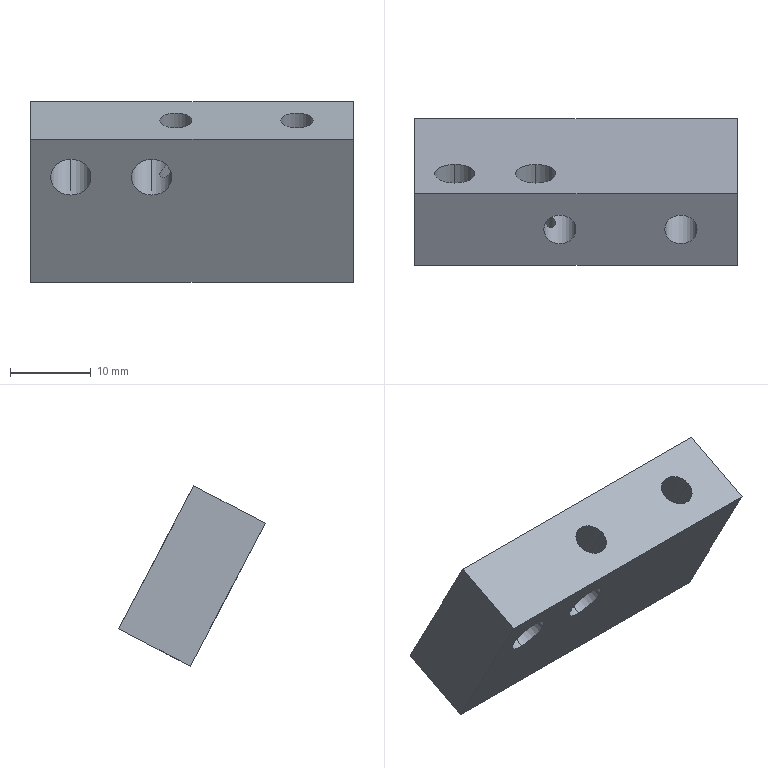Component | SolidWorks | ToolHolderAssembly-1_CutterFixingBlock-1 | 1 solid | 14 faces | box 40 x 18.15 x 22.36 mm | volume 7118 mm3 | cylinder 8 | plane 6 | commonest cylinder face diameters 5 x4 4 x4
build123d program:
from build123d import *

# Parameters (mm, degrees)
SKETCH1_W                = 40
SKETCH1_H                = 10
BOSS_EXTRUDE1_DEPTH      = 20
M4_TAPPED_HOLE1_D        = 4
F_5_0_5_DIAMETER_HOLE1_D = 5


with BuildPart() as part:
    # Sketch1 → Boss-Extrude1 (new body)
    with BuildSketch(Plane.XY):
        Rectangle(SKETCH1_W, SKETCH1_H)
    extrude(amount=BOSS_EXTRUDE1_DEPTH)

    # M4 Tapped Hole1 (through all)
    with Locations(Plane(origin=(0, 0, 0), x_dir=(-1, 0, 0), z_dir=(0, 0, -1))):
        with Locations((13, 0), (-2, 0)):
            Hole(M4_TAPPED_HOLE1_D / 2)

    # 5.0 _5_ Diameter Hole1 (through all)
    with Locations(Plane(origin=(0, 5, 0), x_dir=(1, 0, 0), z_dir=(0, 1, 0))):
        with Locations((5, -14.698), (15, -14.698)):
            Hole(F_5_0_5_DIAMETER_HOLE1_D / 2)


solid = part.part

# Placed as in the assembly
solid = solid.moved(Location((-170.317, -6.727, 164.158), (27.698, 0, 180)))
STEP:
#1=COLOUR_RGB('',0.7922,0.8196,0.9333);
#2=FILL_AREA_STYLE_COLOUR('',#1);
#3=FILL_AREA_STYLE('',(#2));
#4=SURFACE_STYLE_FILL_AREA(#3);
#5=SURFACE_SIDE_STYLE('',(#4));
#6=SURFACE_STYLE_USAGE(.BOTH.,#5);
#7=PRESENTATION_STYLE_ASSIGNMENT((#6));
#8=CARTESIAN_POINT('',(-6.863,-0.5757,7.055));
#9=VERTEX_POINT('',#8);
#10=CARTESIAN_POINT('',(-6.863,-0.4919,6.895));
#11=VERTEX_POINT('',#10);
#12=CARTESIAN_POINT('',(-6.863,-0.5757,7.055));
#13=CARTESIAN_POINT('',(-6.863,-0.57,7.058));
#14=CARTESIAN_POINT('',(-6.862,-0.5642,7.061));
#15=CARTESIAN_POINT('',(-6.859,-0.5524,7.065));
#16=CARTESIAN_POINT('',(-6.857,-0.5466,7.067));
#17=CARTESIAN_POINT('',(-6.851,-0.5353,7.069));
#18=CARTESIAN_POINT('',(-6.847,-0.5298,7.07));
#19=CARTESIAN_POINT('',(-6.84,-0.5194,7.069));
#20=CARTESIAN_POINT('',(-6.835,-0.5145,7.067));
#21=CARTESIAN_POINT('',(-6.828,-0.5054,7.063));
#22=CARTESIAN_POINT('',(-6.824,-0.5011,7.06));
#23=CARTESIAN_POINT('',(-6.817,-0.4931,7.052));
#24=CARTESIAN_POINT('',(-6.814,-0.4894,7.048));
#25=CARTESIAN_POINT('',(-6.809,-0.4823,7.038));
#26=CARTESIAN_POINT('',(-6.807,-0.4789,7.033));
#27=CARTESIAN_POINT('',(-6.804,-0.4724,7.022));
#28=CARTESIAN_POINT('',(-6.804,-0.4693,7.016));
#29=CARTESIAN_POINT('',(-6.804,-0.4603,6.999));
#30=CARTESIAN_POINT('',(-6.806,-0.4547,6.988));
#31=CARTESIAN_POINT('',(-6.814,-0.4489,6.971));
#32=CARTESIAN_POINT('',(-6.817,-0.4474,6.965));
#33=CARTESIAN_POINT('',(-6.824,-0.4457,6.954));
#34=CARTESIAN_POINT('',(-6.827,-0.4456,6.949));
#35=CARTESIAN_POINT('',(-6.835,-0.447,6.939));
#36=CARTESIAN_POINT('',(-6.84,-0.4487,6.934));
#37=CARTESIAN_POINT('',(-6.847,-0.4537,6.925));
#38=CARTESIAN_POINT('',(-6.851,-0.4572,6.921));
#39=CARTESIAN_POINT('',(-6.857,-0.4654,6.913));
#40=CARTESIAN_POINT('',(-6.859,-0.4702,6.909));
#41=CARTESIAN_POINT('',(-6.862,-0.4805,6.902));
#42=CARTESIAN_POINT('',(-6.863,-0.4862,6.898));
#43=CARTESIAN_POINT('',(-6.863,-0.4919,6.895));
#44=B_SPLINE_CURVE_WITH_KNOTS('',3,(#12,#13,#14,#15,#16,#17,#18,#19,#20,#21,#22,#23,#24,#25,#26,#27,#28,#29,#30,#31,#32,#33,#34,#35,#36,#37,#38,#39,#40,#41,#42,#43),.UNSPECIFIED.,.F.,.F.,(4,2,2,2,2,2,2,2,2,2,2,2,2,2,2,4),(0.,0.0004904,0.0009807,0.001471,0.001961,0.002452,0.002942,0.003433,0.003923,0.004904,0.005394,0.005884,0.006375,0.006865,0.007355,0.007846),.UNSPECIFIED.);
#45=EDGE_CURVE('',#9,#11,#44,.T.);
#46=ORIENTED_EDGE('',*,*,#45,.F.);
#47=CARTESIAN_POINT('',(-6.863,-0.4919,6.895));
#48=CARTESIAN_POINT('',(-6.863,-0.4976,6.892));
#49=CARTESIAN_POINT('',(-6.862,-0.5035,6.89));
#50=CARTESIAN_POINT('',(-6.859,-0.5152,6.885));
#51=CARTESIAN_POINT('',(-6.857,-0.521,6.883));
#52=CARTESIAN_POINT('',(-6.851,-0.5323,6.881));
#53=CARTESIAN_POINT('',(-6.847,-0.5378,6.881));
#54=CARTESIAN_POINT('',(-6.84,-0.5482,6.882));
#55=CARTESIAN_POINT('',(-6.835,-0.5531,6.883));
#56=CARTESIAN_POINT('',(-6.828,-0.5622,6.888));
#57=CARTESIAN_POINT('',(-6.824,-0.5665,6.891));
#58=CARTESIAN_POINT('',(-6.817,-0.5744,6.898));
#59=CARTESIAN_POINT('',(-6.814,-0.5782,6.903));
#60=CARTESIAN_POINT('',(-6.806,-0.5888,6.917));
#61=CARTESIAN_POINT('',(-6.804,-0.5953,6.928));
#62=CARTESIAN_POINT('',(-6.804,-0.6043,6.946));
#63=CARTESIAN_POINT('',(-6.804,-0.6072,6.951));
#64=CARTESIAN_POINT('',(-6.807,-0.6124,6.963));
#65=CARTESIAN_POINT('',(-6.809,-0.6148,6.969));
#66=CARTESIAN_POINT('',(-6.814,-0.6187,6.98));
#67=CARTESIAN_POINT('',(-6.817,-0.6202,6.985));
#68=CARTESIAN_POINT('',(-6.824,-0.6219,6.996));
#69=CARTESIAN_POINT('',(-6.827,-0.622,7.001));
#70=CARTESIAN_POINT('',(-6.835,-0.6206,7.012));
#71=CARTESIAN_POINT('',(-6.839,-0.619,7.016));
#72=CARTESIAN_POINT('',(-6.847,-0.6139,7.025));
#73=CARTESIAN_POINT('',(-6.851,-0.6105,7.03));
#74=CARTESIAN_POINT('',(-6.857,-0.6023,7.038));
#75=CARTESIAN_POINT('',(-6.859,-0.5975,7.042));
#76=CARTESIAN_POINT('',(-6.862,-0.5871,7.049));
#77=CARTESIAN_POINT('',(-6.863,-0.5815,7.052));
#78=CARTESIAN_POINT('',(-6.863,-0.5757,7.055));
#79=B_SPLINE_CURVE_WITH_KNOTS('',3,(#47,#48,#49,#50,#51,#52,#53,#54,#55,#56,#57,#58,#59,#60,#61,#62,#63,#64,#65,#66,#67,#68,#69,#70,#71,#72,#73,#74,#75,#76,#77,#78),.UNSPECIFIED.,.F.,.F.,(4,2,2,2,2,2,2,2,2,2,2,2,2,2,2,4),(0.007846,0.008336,0.008826,0.009316,0.009805,0.0103,0.01079,0.01177,0.01225,0.01274,0.01323,0.01372,0.01421,0.0147,0.01519,0.01568),.UNSPECIFIED.);
#80=EDGE_CURVE('',#11,#9,#79,.T.);
#81=ORIENTED_EDGE('',*,*,#80,.F.);
#82=EDGE_LOOP('',(#46,#81));
#83=FACE_BOUND('',#82,.T.);
#84=CARTESIAN_POINT('',(-6.902,-0.3138,6.98));
#85=VERTEX_POINT('',#84);
#86=CARTESIAN_POINT('',(-6.902,-0.4053,7.154));
#87=VERTEX_POINT('',#86);
#88=CARTESIAN_POINT('',(-6.902,-0.3595,7.067));
#89=DIRECTION('',(0.,-0.8854,-0.4648));
#90=DIRECTION('',(-0.,-0.4648,0.8854));
#91=AXIS2_PLACEMENT_3D('',#88,#89,#90);
#92=CIRCLE('',#91,0.09843);
#93=EDGE_CURVE('',#85,#87,#92,.T.);
#94=ORIENTED_EDGE('',*,*,#93,.F.);
#95=CARTESIAN_POINT('',(-6.902,-0.6623,6.797));
#96=VERTEX_POINT('',#95);
#97=CARTESIAN_POINT('',(-6.902,-0.6623,6.797));
#98=DIRECTION('',(0.,-0.8854,-0.4648));
#99=VECTOR('',#98,39.37);
#100=LINE('',#97,#99);
#101=EDGE_CURVE('',#85,#96,#100,.T.);
#102=ORIENTED_EDGE('',*,*,#101,.T.);
#103=CARTESIAN_POINT('',(-6.902,-0.7538,6.971));
#104=VERTEX_POINT('',#103);
#105=CARTESIAN_POINT('',(-6.902,-0.7081,6.884));
#106=DIRECTION('',(0.,-0.8854,-0.4648));
#107=DIRECTION('',(-0.,-0.4648,0.8854));
#108=AXIS2_PLACEMENT_3D('',#105,#106,#107);
#109=CIRCLE('',#108,0.09843);
#110=EDGE_CURVE('',#96,#104,#109,.T.);
#111=ORIENTED_EDGE('',*,*,#110,.T.);
#112=CARTESIAN_POINT('',(-6.902,-0.7538,6.971));
#113=DIRECTION('',(0.,-0.8854,-0.4648));
#114=VECTOR('',#113,39.37);
#115=LINE('',#112,#114);
#116=EDGE_CURVE('',#87,#104,#115,.T.);
#117=ORIENTED_EDGE('',*,*,#116,.F.);
#118=EDGE_LOOP('',(#94,#102,#111,#117));
#119=FACE_OUTER_BOUND('',#118,.T.);
#120=CARTESIAN_POINT('',(-6.902,-0.7081,6.884));
#121=DIRECTION('',(0.,-0.8854,-0.4648));
#122=DIRECTION('',(-0.,-0.4648,0.8854));
#123=AXIS2_PLACEMENT_3D('',#120,#121,#122);
#124=CYLINDRICAL_SURFACE('',#123,0.09843);
#125=ADVANCED_FACE('',(#83,#119),#124,.F.);
#126=CARTESIAN_POINT('',(-7.296,-0.3138,6.98));
#127=VERTEX_POINT('',#126);
#128=CARTESIAN_POINT('',(-7.296,-0.4053,7.154));
#129=VERTEX_POINT('',#128);
#130=CARTESIAN_POINT('',(-7.296,-0.3595,7.067));
#131=DIRECTION('',(0.,-0.8854,-0.4648));
#132=DIRECTION('',(-0.,-0.4648,0.8854));
#133=AXIS2_PLACEMENT_3D('',#130,#131,#132);
#134=CIRCLE('',#133,0.09843);
#135=EDGE_CURVE('',#127,#129,#134,.T.);
#136=ORIENTED_EDGE('',*,*,#135,.F.);
#137=CARTESIAN_POINT('',(-7.296,-0.6623,6.797));
#138=VERTEX_POINT('',#137);
#139=CARTESIAN_POINT('',(-7.296,-0.6623,6.797));
#140=DIRECTION('',(0.,-0.8854,-0.4648));
#141=VECTOR('',#140,39.37);
#142=LINE('',#139,#141);
#143=EDGE_CURVE('',#127,#138,#142,.T.);
#144=ORIENTED_EDGE('',*,*,#143,.T.);
#145=CARTESIAN_POINT('',(-7.296,-0.7538,6.971));
#146=VERTEX_POINT('',#145);
#147=CARTESIAN_POINT('',(-7.296,-0.7081,6.884));
#148=DIRECTION('',(0.,-0.8854,-0.4648));
#149=DIRECTION('',(-0.,-0.4648,0.8854));
#150=AXIS2_PLACEMENT_3D('',#147,#148,#149);
#151=CIRCLE('',#150,0.09843);
#152=EDGE_CURVE('',#138,#146,#151,.T.);
#153=ORIENTED_EDGE('',*,*,#152,.T.);
#154=CARTESIAN_POINT('',(-7.296,-0.7538,6.971));
#155=DIRECTION('',(0.,-0.8854,-0.4648));
#156=VECTOR('',#155,39.37);
#157=LINE('',#154,#156);
#158=EDGE_CURVE('',#129,#146,#157,.T.);
#159=ORIENTED_EDGE('',*,*,#158,.F.);
#160=EDGE_LOOP('',(#136,#144,#153,#159));
#161=FACE_OUTER_BOUND('',#160,.T.);
#162=CARTESIAN_POINT('',(-7.296,-0.7081,6.884));
#163=DIRECTION('',(0.,-0.8854,-0.4648));
#164=DIRECTION('',(-0.,-0.4648,0.8854));
#165=AXIS2_PLACEMENT_3D('',#162,#163,#164);
#166=CYLINDRICAL_SURFACE('',#165,0.09843);
#167=ADVANCED_FACE('',(#161),#166,.F.);
#168=CARTESIAN_POINT('',(-6.272,-0.6308,7.16));
#169=VERTEX_POINT('',#168);
#170=CARTESIAN_POINT('',(-6.115,-0.6308,7.16));
#171=VERTEX_POINT('',#170);
#172=CARTESIAN_POINT('',(-6.194,-0.6308,7.16));
#173=DIRECTION('',(0.,0.4648,-0.8854));
#174=DIRECTION('',(1.,-0.,0.));
#175=AXIS2_PLACEMENT_3D('',#172,#173,#174);
#176=CIRCLE('',#175,0.07874);
#177=EDGE_CURVE('',#169,#171,#176,.T.);
#178=ORIENTED_EDGE('',*,*,#177,.F.);
#179=CARTESIAN_POINT('',(-6.272,-0.2648,6.463));
#180=VERTEX_POINT('',#179);
#181=CARTESIAN_POINT('',(-6.272,-0.2648,6.463));
#182=DIRECTION('',(0.,0.4648,-0.8854));
#183=VECTOR('',#182,39.37);
#184=LINE('',#181,#183);
#185=EDGE_CURVE('',#169,#180,#184,.T.);
#186=ORIENTED_EDGE('',*,*,#185,.T.);
#187=CARTESIAN_POINT('',(-6.115,-0.2648,6.463));
#188=VERTEX_POINT('',#187);
#189=CARTESIAN_POINT('',(-6.194,-0.2648,6.463));
#190=DIRECTION('',(0.,0.4648,-0.8854));
#191=DIRECTION('',(1.,-0.,0.));
#192=AXIS2_PLACEMENT_3D('',#189,#190,#191);
#193=CIRCLE('',#192,0.07874);
#194=EDGE_CURVE('',#180,#188,#193,.T.);
#195=ORIENTED_EDGE('',*,*,#194,.T.);
#196=CARTESIAN_POINT('',(-6.115,-0.2648,6.463));
#197=DIRECTION('',(0.,0.4648,-0.8854));
#198=VECTOR('',#197,39.37);
#199=LINE('',#196,#198);
#200=EDGE_CURVE('',#171,#188,#199,.T.);
#201=ORIENTED_EDGE('',*,*,#200,.F.);
#202=EDGE_LOOP('',(#178,#186,#195,#201));
#203=FACE_OUTER_BOUND('',#202,.T.);
#204=CARTESIAN_POINT('',(-6.194,-0.2648,6.463));
#205=DIRECTION('',(0.,0.4648,-0.8854));
#206=DIRECTION('',(1.,-0.,0.));
#207=AXIS2_PLACEMENT_3D('',#204,#205,#206);
#208=CYLINDRICAL_SURFACE('',#207,0.07874);
#209=ADVANCED_FACE('',(#203),#208,.F.);
#210=CARTESIAN_POINT('',(-6.863,-0.6308,7.16));
#211=VERTEX_POINT('',#210);
#212=CARTESIAN_POINT('',(-6.705,-0.6308,7.16));
#213=VERTEX_POINT('',#212);
#214=CARTESIAN_POINT('',(-6.784,-0.6308,7.16));
#215=DIRECTION('',(0.,0.4648,-0.8854));
#216=DIRECTION('',(1.,-0.,0.));
#217=AXIS2_PLACEMENT_3D('',#214,#215,#216);
#218=CIRCLE('',#217,0.07874);
#219=EDGE_CURVE('',#211,#213,#218,.T.);
#220=ORIENTED_EDGE('',*,*,#219,.F.);
#221=CARTESIAN_POINT('',(-6.863,-0.2648,6.463));
#222=DIRECTION('',(0.,0.4648,-0.8854));
#223=VECTOR('',#222,39.37);
#224=LINE('',#221,#223);
#225=EDGE_CURVE('',#211,#9,#224,.T.);
#226=ORIENTED_EDGE('',*,*,#225,.T.);
#227=ORIENTED_EDGE('',*,*,#45,.T.);
#228=CARTESIAN_POINT('',(-6.863,-0.2648,6.463));
#229=VERTEX_POINT('',#228);
#230=CARTESIAN_POINT('',(-6.863,-0.2648,6.463));
#231=DIRECTION('',(0.,0.4648,-0.8854));
#232=VECTOR('',#231,39.37);
#233=LINE('',#230,#232);
#234=EDGE_CURVE('',#11,#229,#233,.T.);
#235=ORIENTED_EDGE('',*,*,#234,.T.);
#236=CARTESIAN_POINT('',(-6.705,-0.2648,6.463));
#237=VERTEX_POINT('',#236);
#238=CARTESIAN_POINT('',(-6.784,-0.2648,6.463));
#239=DIRECTION('',(0.,0.4648,-0.8854));
#240=DIRECTION('',(1.,-0.,0.));
#241=AXIS2_PLACEMENT_3D('',#238,#239,#240);
#242=CIRCLE('',#241,0.07874);
#243=EDGE_CURVE('',#229,#237,#242,.T.);
#244=ORIENTED_EDGE('',*,*,#243,.T.);
#245=CARTESIAN_POINT('',(-6.705,-0.2648,6.463));
#246=DIRECTION('',(0.,0.4648,-0.8854));
#247=VECTOR('',#246,39.37);
#248=LINE('',#245,#247);
#249=EDGE_CURVE('',#213,#237,#248,.T.);
#250=ORIENTED_EDGE('',*,*,#249,.F.);
#251=EDGE_LOOP('',(#220,#226,#227,#235,#244,#250));
#252=FACE_OUTER_BOUND('',#251,.T.);
#253=CARTESIAN_POINT('',(-6.784,-0.2648,6.463));
#254=DIRECTION('',(0.,0.4648,-0.8854));
#255=DIRECTION('',(1.,-0.,0.));
#256=AXIS2_PLACEMENT_3D('',#253,#254,#255);
#257=CYLINDRICAL_SURFACE('',#256,0.07874);
#258=ADVANCED_FACE('',(#252),#257,.F.);
#259=CARTESIAN_POINT('',(-7.493,-0.09053,6.554));
#260=VERTEX_POINT('',#259);
#261=CARTESIAN_POINT('',(-7.493,-0.4391,6.371));
#262=VERTEX_POINT('',#261);
#263=CARTESIAN_POINT('',(-7.493,-0.09053,6.554));
#264=DIRECTION('',(0.,-0.8854,-0.4648));
#265=VECTOR('',#264,39.37);
#266=LINE('',#263,#265);
#267=EDGE_CURVE('',#260,#262,#266,.T.);
#268=ORIENTED_EDGE('',*,*,#267,.T.);
#269=CARTESIAN_POINT('',(-7.493,-0.8051,7.069));
#270=VERTEX_POINT('',#269);
#271=CARTESIAN_POINT('',(-7.493,-0.8051,7.069));
#272=DIRECTION('',(0.,0.4648,-0.8854));
#273=VECTOR('',#272,39.37);
#274=LINE('',#271,#273);
#275=EDGE_CURVE('',#270,#262,#274,.T.);
#276=ORIENTED_EDGE('',*,*,#275,.F.);
#277=CARTESIAN_POINT('',(-7.493,-0.4565,7.252));
#278=VERTEX_POINT('',#277);
#279=CARTESIAN_POINT('',(-7.493,-0.4565,7.252));
#280=DIRECTION('',(0.,-0.8854,-0.4648));
#281=VECTOR('',#280,39.37);
#282=LINE('',#279,#281);
#283=EDGE_CURVE('',#278,#270,#282,.T.);
#284=ORIENTED_EDGE('',*,*,#283,.F.);
#285=CARTESIAN_POINT('',(-7.493,-0.4565,7.252));
#286=DIRECTION('',(0.,0.4648,-0.8854));
#287=VECTOR('',#286,39.37);
#288=LINE('',#285,#287);
#289=EDGE_CURVE('',#278,#260,#288,.T.);
#290=ORIENTED_EDGE('',*,*,#289,.T.);
#291=EDGE_LOOP('',(#268,#276,#284,#290));
#292=FACE_OUTER_BOUND('',#291,.T.);
#293=CARTESIAN_POINT('',(-7.493,-0.4565,7.252));
#294=DIRECTION('',(1.,-0.,0.));
#295=DIRECTION('',(-0.,-0.4648,0.8854));
#296=AXIS2_PLACEMENT_3D('',#293,#294,#295);
#297=PLANE('',#296);
#298=ADVANCED_FACE('',(#292),#297,.F.);
#299=CARTESIAN_POINT('',(-6.902,-0.7081,6.884));
#300=DIRECTION('',(0.,-0.8854,-0.4648));
#301=DIRECTION('',(-0.,-0.4648,0.8854));
#302=AXIS2_PLACEMENT_3D('',#299,#300,#301);
#303=CIRCLE('',#302,0.09843);
#304=EDGE_CURVE('',#104,#96,#303,.T.);
#305=ORIENTED_EDGE('',*,*,#304,.F.);
#306=ORIENTED_EDGE('',*,*,#110,.F.);
#307=EDGE_LOOP('',(#305,#306));
#308=FACE_BOUND('',#307,.T.);
#309=CARTESIAN_POINT('',(-7.296,-0.7081,6.884));
#310=DIRECTION('',(0.,-0.8854,-0.4648));
#311=DIRECTION('',(-0.,-0.4648,0.8854));
#312=AXIS2_PLACEMENT_3D('',#309,#310,#311);
#313=CIRCLE('',#312,0.09843);
#314=EDGE_CURVE('',#146,#138,#313,.T.);
#315=ORIENTED_EDGE('',*,*,#314,.F.);
#316=ORIENTED_EDGE('',*,*,#152,.F.);
#317=EDGE_LOOP('',(#315,#316));
#318=FACE_BOUND('',#317,.T.);
#319=CARTESIAN_POINT('',(-5.918,-0.4391,6.371));
#320=VERTEX_POINT('',#319);
#321=CARTESIAN_POINT('',(-5.918,-0.4391,6.371));
#322=DIRECTION('',(1.,-0.,0.));
#323=VECTOR('',#322,39.37);
#324=LINE('',#321,#323);
#325=EDGE_CURVE('',#262,#320,#324,.T.);
#326=ORIENTED_EDGE('',*,*,#325,.T.);
#327=CARTESIAN_POINT('',(-5.918,-0.8051,7.069));
#328=VERTEX_POINT('',#327);
#329=CARTESIAN_POINT('',(-5.918,-0.8051,7.069));
#330=DIRECTION('',(0.,0.4648,-0.8854));
#331=VECTOR('',#330,39.37);
#332=LINE('',#329,#331);
#333=EDGE_CURVE('',#328,#320,#332,.T.);
#334=ORIENTED_EDGE('',*,*,#333,.F.);
#335=CARTESIAN_POINT('',(-5.918,-0.8051,7.069));
#336=DIRECTION('',(1.,-0.,0.));
#337=VECTOR('',#336,39.37);
#338=LINE('',#335,#337);
#339=EDGE_CURVE('',#270,#328,#338,.T.);
#340=ORIENTED_EDGE('',*,*,#339,.F.);
#341=ORIENTED_EDGE('',*,*,#275,.T.);
#342=EDGE_LOOP('',(#326,#334,#340,#341));
#343=FACE_OUTER_BOUND('',#342,.T.);
#344=CARTESIAN_POINT('',(-5.918,-0.8051,7.069));
#345=DIRECTION('',(-0.,0.8854,0.4648));
#346=DIRECTION('',(0.,0.4648,-0.8854));
#347=AXIS2_PLACEMENT_3D('',#344,#345,#346);
#348=PLANE('',#347);
#349=ADVANCED_FACE('',(#308,#318,#343),#348,.F.);
#350=CARTESIAN_POINT('',(-5.918,-0.09053,6.554));
#351=VERTEX_POINT('',#350);
#352=CARTESIAN_POINT('',(-5.918,-0.09053,6.554));
#353=DIRECTION('',(-0.,0.8854,0.4648));
#354=VECTOR('',#353,39.37);
#355=LINE('',#352,#354);
#356=EDGE_CURVE('',#320,#351,#355,.T.);
#357=ORIENTED_EDGE('',*,*,#356,.T.);
#358=CARTESIAN_POINT('',(-5.918,-0.4565,7.252));
#359=VERTEX_POINT('',#358);
#360=CARTESIAN_POINT('',(-5.918,-0.4565,7.252));
#361=DIRECTION('',(0.,0.4648,-0.8854));
#362=VECTOR('',#361,39.37);
#363=LINE('',#360,#362);
#364=EDGE_CURVE('',#359,#351,#363,.T.);
#365=ORIENTED_EDGE('',*,*,#364,.F.);
#366=CARTESIAN_POINT('',(-5.918,-0.4565,7.252));
#367=DIRECTION('',(-0.,0.8854,0.4648));
#368=VECTOR('',#367,39.37);
#369=LINE('',#366,#368);
#370=EDGE_CURVE('',#328,#359,#369,.T.);
#371=ORIENTED_EDGE('',*,*,#370,.F.);
#372=ORIENTED_EDGE('',*,*,#333,.T.);
#373=EDGE_LOOP('',(#357,#365,#371,#372));
#374=FACE_OUTER_BOUND('',#373,.T.);
#375=CARTESIAN_POINT('',(-5.918,-0.4565,7.252));
#376=DIRECTION('',(-1.,0.,-0.));
#377=DIRECTION('',(0.,0.4648,-0.8854));
#378=AXIS2_PLACEMENT_3D('',#375,#376,#377);
#379=PLANE('',#378);
#380=ADVANCED_FACE('',(#374),#379,.F.);
#381=CARTESIAN_POINT('',(-6.902,-0.3595,7.067));
#382=DIRECTION('',(0.,-0.8854,-0.4648));
#383=DIRECTION('',(-0.,-0.4648,0.8854));
#384=AXIS2_PLACEMENT_3D('',#381,#382,#383);
#385=CIRCLE('',#384,0.09843);
#386=EDGE_CURVE('',#87,#85,#385,.T.);
#387=ORIENTED_EDGE('',*,*,#386,.T.);
#388=ORIENTED_EDGE('',*,*,#93,.T.);
#389=EDGE_LOOP('',(#387,#388));
#390=FACE_BOUND('',#389,.T.);
#391=CARTESIAN_POINT('',(-7.296,-0.3595,7.067));
#392=DIRECTION('',(0.,-0.8854,-0.4648));
#393=DIRECTION('',(-0.,-0.4648,0.8854));
#394=AXIS2_PLACEMENT_3D('',#391,#392,#393);
#395=CIRCLE('',#394,0.09843);
#396=EDGE_CURVE('',#129,#127,#395,.T.);
#397=ORIENTED_EDGE('',*,*,#396,.T.);
#398=ORIENTED_EDGE('',*,*,#135,.T.);
#399=EDGE_LOOP('',(#397,#398));
#400=FACE_BOUND('',#399,.T.);
#401=CARTESIAN_POINT('',(-5.918,-0.09053,6.554));
#402=DIRECTION('',(-1.,0.,-0.));
#403=VECTOR('',#402,39.37);
#404=LINE('',#401,#403);
#405=EDGE_CURVE('',#351,#260,#404,.T.);
#406=ORIENTED_EDGE('',*,*,#405,.T.);
#407=ORIENTED_EDGE('',*,*,#289,.F.);
#408=CARTESIAN_POINT('',(-5.918,-0.4565,7.252));
#409=DIRECTION('',(-1.,0.,-0.));
#410=VECTOR('',#409,39.37);
#411=LINE('',#408,#410);
#412=EDGE_CURVE('',#359,#278,#411,.T.);
#413=ORIENTED_EDGE('',*,*,#412,.F.);
#414=ORIENTED_EDGE('',*,*,#364,.T.);
#415=EDGE_LOOP('',(#406,#407,#413,#414));
#416=FACE_OUTER_BOUND('',#415,.T.);
#417=CARTESIAN_POINT('',(-5.918,-0.4565,7.252));
#418=DIRECTION('',(0.,-0.8854,-0.4648));
#419=DIRECTION('',(-0.,-0.4648,0.8854));
#420=AXIS2_PLACEMENT_3D('',#417,#418,#419);
#421=PLANE('',#420);
#422=ADVANCED_FACE('',(#390,#400,#416),#421,.F.);
#423=CARTESIAN_POINT('',(-6.194,-0.6308,7.16));
#424=DIRECTION('',(0.,0.4648,-0.8854));
#425=DIRECTION('',(1.,-0.,0.));
#426=AXIS2_PLACEMENT_3D('',#423,#424,#425);
#427=CIRCLE('',#426,0.07874);
#428=EDGE_CURVE('',#171,#169,#427,.T.);
#429=ORIENTED_EDGE('',*,*,#428,.T.);
#430=ORIENTED_EDGE('',*,*,#177,.T.);
#431=EDGE_LOOP('',(#429,#430));
#432=FACE_BOUND('',#431,.T.);
#433=CARTESIAN_POINT('',(-6.784,-0.6308,7.16));
#434=DIRECTION('',(0.,0.4648,-0.8854));
#435=DIRECTION('',(1.,-0.,0.));
#436=AXIS2_PLACEMENT_3D('',#433,#434,#435);
#437=CIRCLE('',#436,0.07874);
#438=EDGE_CURVE('',#213,#211,#437,.T.);
#439=ORIENTED_EDGE('',*,*,#438,.T.);
#440=ORIENTED_EDGE('',*,*,#219,.T.);
#441=EDGE_LOOP('',(#439,#440));
#442=FACE_BOUND('',#441,.T.);
#443=ORIENTED_EDGE('',*,*,#283,.T.);
#444=ORIENTED_EDGE('',*,*,#339,.T.);
#445=ORIENTED_EDGE('',*,*,#370,.T.);
#446=ORIENTED_EDGE('',*,*,#412,.T.);
#447=EDGE_LOOP('',(#443,#444,#445,#446));
#448=FACE_OUTER_BOUND('',#447,.T.);
#449=CARTESIAN_POINT('',(-6.705,-0.6308,7.16));
#450=DIRECTION('',(0.,0.4648,-0.8854));
#451=DIRECTION('',(1.,-0.,0.));
#452=AXIS2_PLACEMENT_3D('',#449,#450,#451);
#453=PLANE('',#452);
#454=ADVANCED_FACE('',(#432,#442,#448),#453,.F.);
#455=CARTESIAN_POINT('',(-6.194,-0.2648,6.463));
#456=DIRECTION('',(0.,0.4648,-0.8854));
#457=DIRECTION('',(1.,-0.,0.));
#458=AXIS2_PLACEMENT_3D('',#455,#456,#457);
#459=CIRCLE('',#458,0.07874);
#460=EDGE_CURVE('',#188,#180,#459,.T.);
#461=ORIENTED_EDGE('',*,*,#460,.F.);
#462=ORIENTED_EDGE('',*,*,#194,.F.);
#463=EDGE_LOOP('',(#461,#462));
#464=FACE_BOUND('',#463,.T.);
#465=CARTESIAN_POINT('',(-6.784,-0.2648,6.463));
#466=DIRECTION('',(0.,0.4648,-0.8854));
#467=DIRECTION('',(1.,-0.,0.));
#468=AXIS2_PLACEMENT_3D('',#465,#466,#467);
#469=CIRCLE('',#468,0.07874);
#470=EDGE_CURVE('',#237,#229,#469,.T.);
#471=ORIENTED_EDGE('',*,*,#470,.F.);
#472=ORIENTED_EDGE('',*,*,#243,.F.);
#473=EDGE_LOOP('',(#471,#472));
#474=FACE_BOUND('',#473,.T.);
#475=ORIENTED_EDGE('',*,*,#267,.F.);
#476=ORIENTED_EDGE('',*,*,#405,.F.);
#477=ORIENTED_EDGE('',*,*,#356,.F.);
#478=ORIENTED_EDGE('',*,*,#325,.F.);
#479=EDGE_LOOP('',(#475,#476,#477,#478));
#480=FACE_OUTER_BOUND('',#479,.T.);
#481=CARTESIAN_POINT('',(-6.705,-0.2648,6.463));
#482=DIRECTION('',(0.,0.4648,-0.8854));
#483=DIRECTION('',(1.,-0.,0.));
#484=AXIS2_PLACEMENT_3D('',#481,#482,#483);
#485=PLANE('',#484);
#486=ADVANCED_FACE('',(#464,#474,#480),#485,.T.);
#487=ORIENTED_EDGE('',*,*,#225,.F.);
#488=ORIENTED_EDGE('',*,*,#438,.F.);
#489=ORIENTED_EDGE('',*,*,#249,.T.);
#490=ORIENTED_EDGE('',*,*,#470,.T.);
#491=ORIENTED_EDGE('',*,*,#234,.F.);
#492=ORIENTED_EDGE('',*,*,#80,.T.);
#493=EDGE_LOOP('',(#487,#488,#489,#490,#491,#492));
#494=FACE_OUTER_BOUND('',#493,.T.);
#495=CARTESIAN_POINT('',(-6.784,-0.2648,6.463));
#496=DIRECTION('',(0.,0.4648,-0.8854));
#497=DIRECTION('',(1.,-0.,0.));
#498=AXIS2_PLACEMENT_3D('',#495,#496,#497);
#499=CYLINDRICAL_SURFACE('',#498,0.07874);
#500=ADVANCED_FACE('',(#494),#499,.F.);
#501=ORIENTED_EDGE('',*,*,#185,.F.);
#502=ORIENTED_EDGE('',*,*,#428,.F.);
#503=ORIENTED_EDGE('',*,*,#200,.T.);
#504=ORIENTED_EDGE('',*,*,#460,.T.);
#505=EDGE_LOOP('',(#501,#502,#503,#504));
#506=FACE_OUTER_BOUND('',#505,.T.);
#507=CARTESIAN_POINT('',(-6.194,-0.2648,6.463));
#508=DIRECTION('',(0.,0.4648,-0.8854));
#509=DIRECTION('',(1.,-0.,0.));
#510=AXIS2_PLACEMENT_3D('',#507,#508,#509);
#511=CYLINDRICAL_SURFACE('',#510,0.07874);
#512=ADVANCED_FACE('',(#506),#511,.F.);
#513=ORIENTED_EDGE('',*,*,#143,.F.);
#514=ORIENTED_EDGE('',*,*,#396,.F.);
#515=ORIENTED_EDGE('',*,*,#158,.T.);
#516=ORIENTED_EDGE('',*,*,#314,.T.);
#517=EDGE_LOOP('',(#513,#514,#515,#516));
#518=FACE_OUTER_BOUND('',#517,.T.);
#519=CARTESIAN_POINT('',(-7.296,-0.7081,6.884));
#520=DIRECTION('',(0.,-0.8854,-0.4648));
#521=DIRECTION('',(-0.,-0.4648,0.8854));
#522=AXIS2_PLACEMENT_3D('',#519,#520,#521);
#523=CYLINDRICAL_SURFACE('',#522,0.09843);
#524=ADVANCED_FACE('',(#518),#523,.F.);
#525=ORIENTED_EDGE('',*,*,#101,.F.);
#526=ORIENTED_EDGE('',*,*,#386,.F.);
#527=ORIENTED_EDGE('',*,*,#116,.T.);
#528=ORIENTED_EDGE('',*,*,#304,.T.);
#529=EDGE_LOOP('',(#525,#526,#527,#528));
#530=FACE_OUTER_BOUND('',#529,.T.);
#531=CARTESIAN_POINT('',(-6.902,-0.7081,6.884));
#532=DIRECTION('',(0.,-0.8854,-0.4648));
#533=DIRECTION('',(-0.,-0.4648,0.8854));
#534=AXIS2_PLACEMENT_3D('',#531,#532,#533);
#535=CYLINDRICAL_SURFACE('',#534,0.09843);
#536=ADVANCED_FACE('',(#530),#535,.F.);
#537=CLOSED_SHELL('',(#125,#167,#209,#258,#298,#349,#380,#422,#454,#486,#500,#512,#524,#536));
#538=MANIFOLD_SOLID_BREP('',#537);
#539=STYLED_ITEM('',(#7),#538);
#540=PRESENTATION_LAYER_ASSIGNMENT('','',(#539));
#541=CARTESIAN_POINT('',(0.,0.,0.));
#542=DIRECTION('',(0.,0.,1.));
#543=DIRECTION('',(1.,0.,0.));
#544=AXIS2_PLACEMENT_3D('',#541,#542,#543);
#545=(LENGTH_UNIT()NAMED_UNIT(*)SI_UNIT($,.METRE.));
#546=LENGTH_MEASURE_WITH_UNIT(LENGTH_MEASURE(0.0254),#545);
#547=DIMENSIONAL_EXPONENTS(1.,0.,0.,0.,0.,0.,0.);
#548=(CONVERSION_BASED_UNIT('',#546)LENGTH_UNIT()NAMED_UNIT(#547));
#549=UNCERTAINTY_MEASURE_WITH_UNIT(LENGTH_MEASURE(0.00001),#548,'','');
#550=(NAMED_UNIT(*)PLANE_ANGLE_UNIT()SI_UNIT($,.RADIAN.));
#551=(NAMED_UNIT(*)SI_UNIT($,.STERADIAN.)SOLID_ANGLE_UNIT());
#552=(GEOMETRIC_REPRESENTATION_CONTEXT(3)GLOBAL_UNCERTAINTY_ASSIGNED_CONTEXT((#549))GLOBAL_UNIT_ASSIGNED_CONTEXT((#548,#550,#551))REPRESENTATION_CONTEXT('',''));
#553=ADVANCED_BREP_SHAPE_REPRESENTATION('',(#538,#544),#552);
#554=(LENGTH_UNIT()NAMED_UNIT(*)SI_UNIT($,.METRE.));
#555=LENGTH_MEASURE_WITH_UNIT(LENGTH_MEASURE(0.0254),#554);
#556=DIMENSIONAL_EXPONENTS(1.,0.,0.,0.,0.,0.,0.);
#557=(CONVERSION_BASED_UNIT('',#555)LENGTH_UNIT()NAMED_UNIT(#556));
#558=UNCERTAINTY_MEASURE_WITH_UNIT(LENGTH_MEASURE(0.00001),#557,'','');
#559=(NAMED_UNIT(*)PLANE_ANGLE_UNIT()SI_UNIT($,.RADIAN.));
#560=(NAMED_UNIT(*)SI_UNIT($,.STERADIAN.)SOLID_ANGLE_UNIT());
#561=(GEOMETRIC_REPRESENTATION_CONTEXT(3)GLOBAL_UNCERTAINTY_ASSIGNED_CONTEXT((#558))GLOBAL_UNIT_ASSIGNED_CONTEXT((#557,#559,#560))REPRESENTATION_CONTEXT('',''));
#562=MECHANICAL_DESIGN_GEOMETRIC_PRESENTATION_REPRESENTATION('',(#539),#561);